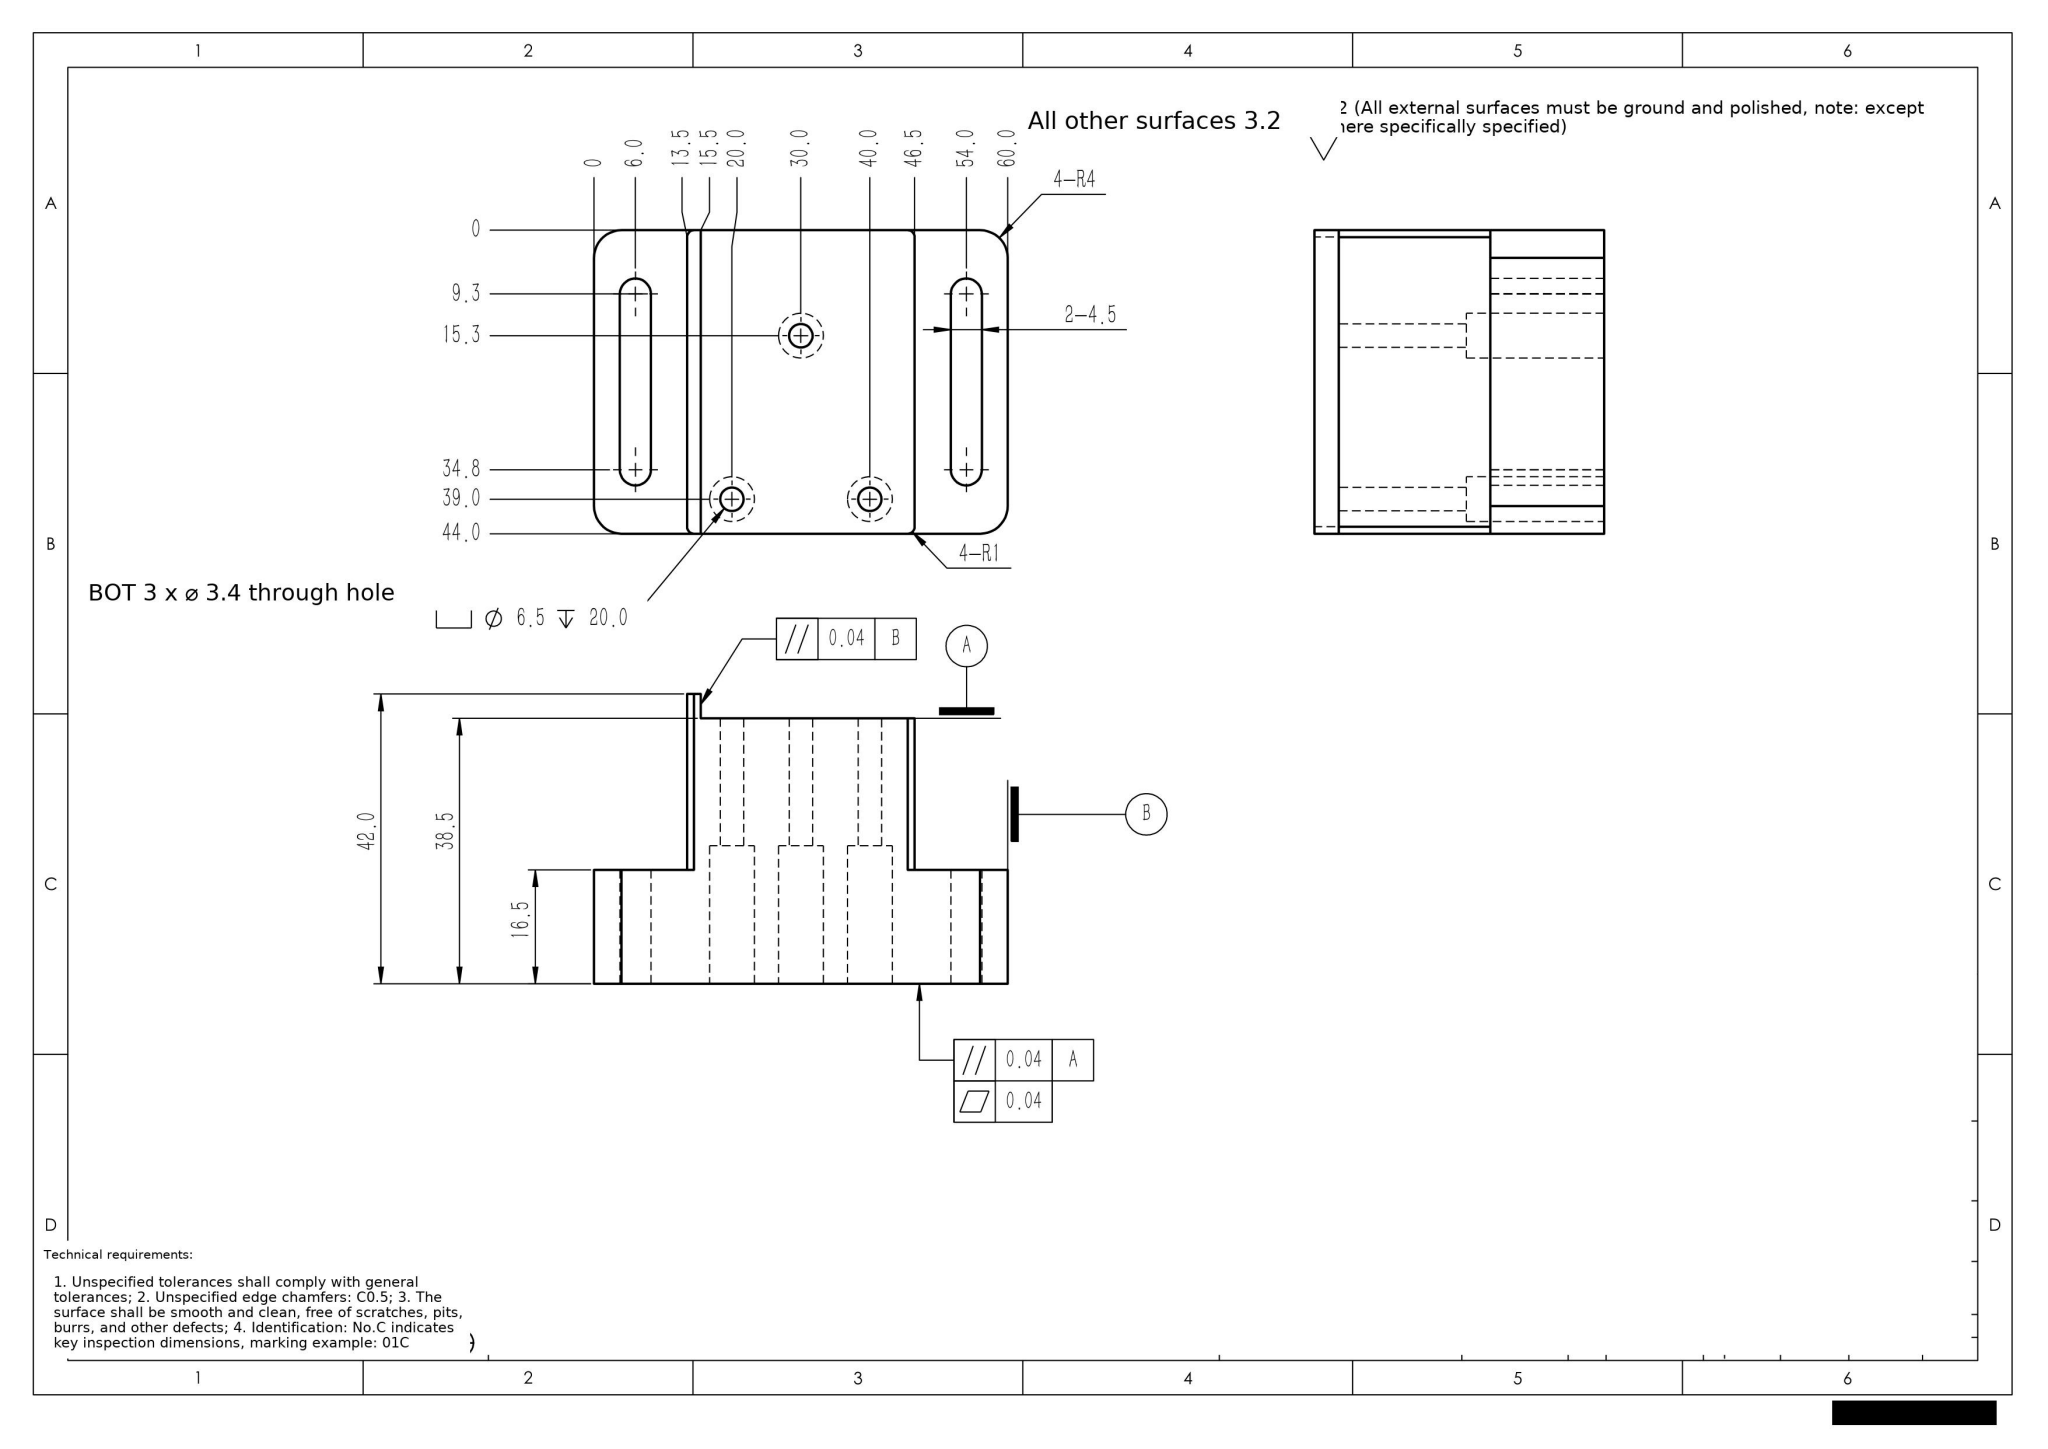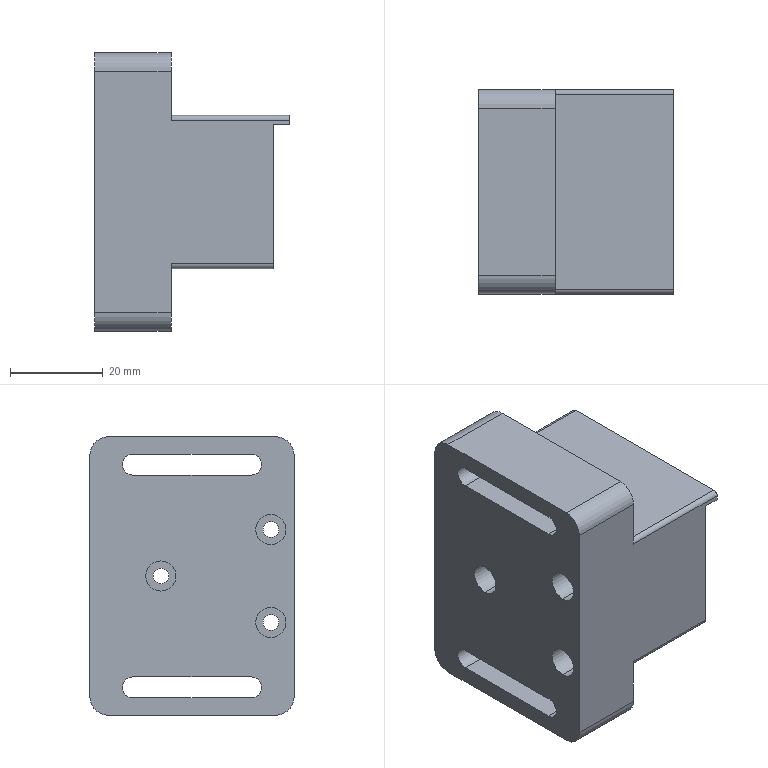Part | SolidWorks | mm | 1 solid | 43 faces | box 42 x 44 x 60 mm | volume 68759 mm3 | cylinder 24 | plane 19 | commonest cylinder face diameters 6.5 x6 3.4 x6 2 x4 8 x4 4.5 x4